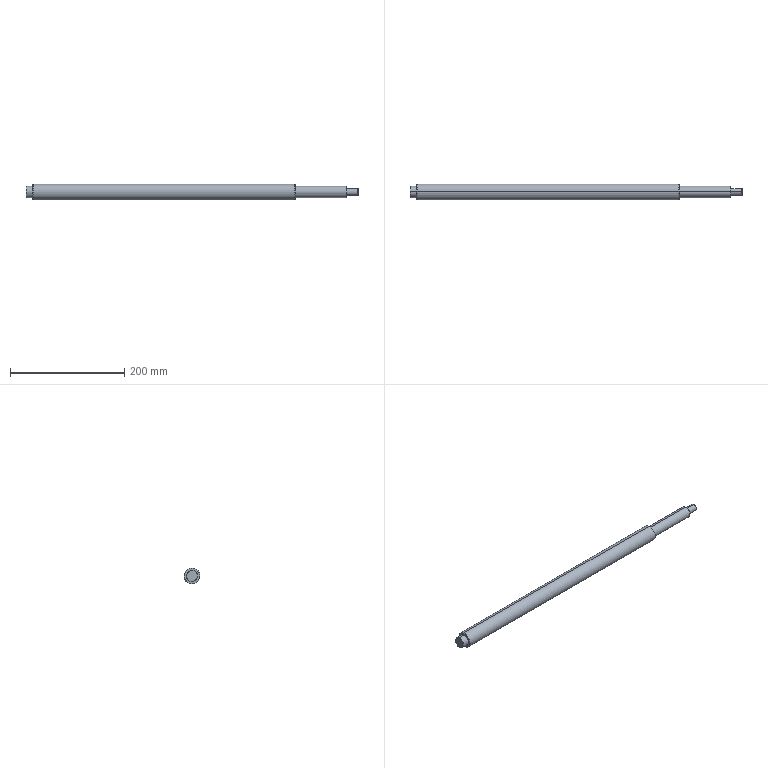Component | SolidWorks | TC020.05-03-1 | 1 solid | 34 faces | box 582 x 28 x 28 mm | volume 317223 mm3 | cone 13 | cylinder 13 | plane 8 | commonest cylinder face diameters 20 x4 12 x3 3.3 x2 28 x2 4 x2 | material 45 Steel
STEP:
#1=COLOUR_RGB('',0.7922,0.8196,0.9333);
#2=FILL_AREA_STYLE_COLOUR('',#1);
#3=FILL_AREA_STYLE('',(#2));
#4=SURFACE_STYLE_FILL_AREA(#3);
#5=SURFACE_SIDE_STYLE('',(#4));
#6=SURFACE_STYLE_USAGE(.BOTH.,#5);
#7=PRESENTATION_STYLE_ASSIGNMENT((#6));
#8=CARTESIAN_POINT('',(0.1969,1.219,0.3721));
#9=VERTEX_POINT('',#8);
#10=CARTESIAN_POINT('',(0.1969,1.143,-0.3721));
#11=VERTEX_POINT('',#10);
#12=CARTESIAN_POINT('',(0.1969,1.181,0.));
#13=DIRECTION('',(-1.,-0.,0.));
#14=DIRECTION('',(0.,0.1006,0.9949));
#15=AXIS2_PLACEMENT_3D('',#12,#13,#14);
#16=CIRCLE('',#15,0.374);
#17=EDGE_CURVE('',#9,#11,#16,.T.);
#18=ORIENTED_EDGE('',*,*,#17,.F.);
#19=CARTESIAN_POINT('',(0.2165,1.221,0.3917));
#20=VERTEX_POINT('',#19);
#21=CARTESIAN_POINT('',(0.2165,1.221,0.3917));
#22=DIRECTION('',(0.7071,0.07111,0.7035));
#23=VECTOR('',#22,39.37);
#24=LINE('',#21,#23);
#25=EDGE_CURVE('',#9,#20,#24,.T.);
#26=ORIENTED_EDGE('',*,*,#25,.T.);
#27=CARTESIAN_POINT('',(0.2165,1.142,-0.3917));
#28=VERTEX_POINT('',#27);
#29=CARTESIAN_POINT('',(0.2165,1.181,0.));
#30=DIRECTION('',(1.,0.,-0.));
#31=DIRECTION('',(0.,0.1006,0.9949));
#32=AXIS2_PLACEMENT_3D('',#29,#30,#31);
#33=CIRCLE('',#32,0.3937);
#34=EDGE_CURVE('',#28,#20,#33,.T.);
#35=ORIENTED_EDGE('',*,*,#34,.F.);
#36=CARTESIAN_POINT('',(0.2165,1.142,-0.3917));
#37=DIRECTION('',(0.7071,-0.07111,-0.7035));
#38=VECTOR('',#37,39.37);
#39=LINE('',#36,#38);
#40=EDGE_CURVE('',#11,#28,#39,.T.);
#41=ORIENTED_EDGE('',*,*,#40,.F.);
#42=EDGE_LOOP('',(#18,#26,#35,#41));
#43=FACE_OUTER_BOUND('',#42,.T.);
#44=CARTESIAN_POINT('',(0.2165,1.181,0.));
#45=DIRECTION('',(1.,0.,-0.));
#46=DIRECTION('',(-0.,-0.1006,-0.9949));
#47=AXIS2_PLACEMENT_3D('',#44,#45,#46);
#48=CONICAL_SURFACE('',#47,0.3937,0.7854);
#49=ADVANCED_FACE('',(#43),#48,.T.);
#50=CARTESIAN_POINT('',(0.6693,1.235,0.5288));
#51=VERTEX_POINT('',#50);
#52=CARTESIAN_POINT('',(0.6693,1.128,-0.5288));
#53=VERTEX_POINT('',#52);
#54=CARTESIAN_POINT('',(0.6693,1.181,0.));
#55=DIRECTION('',(-1.,-0.,0.));
#56=DIRECTION('',(0.,0.1006,0.9949));
#57=AXIS2_PLACEMENT_3D('',#54,#55,#56);
#58=CIRCLE('',#57,0.5315);
#59=EDGE_CURVE('',#51,#53,#58,.T.);
#60=ORIENTED_EDGE('',*,*,#59,.F.);
#61=CARTESIAN_POINT('',(0.689,1.237,0.5484));
#62=VERTEX_POINT('',#61);
#63=CARTESIAN_POINT('',(0.689,1.237,0.5484));
#64=DIRECTION('',(0.7071,0.07111,0.7035));
#65=VECTOR('',#64,39.37);
#66=LINE('',#63,#65);
#67=EDGE_CURVE('',#51,#62,#66,.T.);
#68=ORIENTED_EDGE('',*,*,#67,.T.);
#69=CARTESIAN_POINT('',(0.689,1.126,-0.5484));
#70=VERTEX_POINT('',#69);
#71=CARTESIAN_POINT('',(0.689,1.181,0.));
#72=DIRECTION('',(1.,0.,-0.));
#73=DIRECTION('',(0.,0.1006,0.9949));
#74=AXIS2_PLACEMENT_3D('',#71,#72,#73);
#75=CIRCLE('',#74,0.5512);
#76=EDGE_CURVE('',#70,#62,#75,.T.);
#77=ORIENTED_EDGE('',*,*,#76,.F.);
#78=CARTESIAN_POINT('',(0.689,1.126,-0.5484));
#79=DIRECTION('',(0.7071,-0.07111,-0.7035));
#80=VECTOR('',#79,39.37);
#81=LINE('',#78,#80);
#82=EDGE_CURVE('',#53,#70,#81,.T.);
#83=ORIENTED_EDGE('',*,*,#82,.F.);
#84=EDGE_LOOP('',(#60,#68,#77,#83));
#85=FACE_OUTER_BOUND('',#84,.T.);
#86=CARTESIAN_POINT('',(0.689,1.181,0.));
#87=DIRECTION('',(1.,0.,-0.));
#88=DIRECTION('',(0.,-0.1006,-0.9949));
#89=AXIS2_PLACEMENT_3D('',#86,#87,#88);
#90=CONICAL_SURFACE('',#89,0.5512,0.7854);
#91=ADVANCED_FACE('',(#85),#90,.T.);
#92=CARTESIAN_POINT('',(22.323,1.143,-0.3721));
#93=VERTEX_POINT('',#92);
#94=CARTESIAN_POINT('',(22.323,1.219,0.3721));
#95=VERTEX_POINT('',#94);
#96=CARTESIAN_POINT('',(22.323,1.181,-0.));
#97=DIRECTION('',(1.,0.,-0.));
#98=DIRECTION('',(0.,-0.1006,-0.9949));
#99=AXIS2_PLACEMENT_3D('',#96,#97,#98);
#100=CIRCLE('',#99,0.374);
#101=EDGE_CURVE('',#93,#95,#100,.T.);
#102=ORIENTED_EDGE('',*,*,#101,.F.);
#103=CARTESIAN_POINT('',(22.303,1.142,-0.3917));
#104=VERTEX_POINT('',#103);
#105=CARTESIAN_POINT('',(22.323,1.143,-0.3721));
#106=DIRECTION('',(-0.7071,-0.07111,-0.7035));
#107=VECTOR('',#106,39.37);
#108=LINE('',#105,#107);
#109=EDGE_CURVE('',#93,#104,#108,.T.);
#110=ORIENTED_EDGE('',*,*,#109,.T.);
#111=CARTESIAN_POINT('',(22.303,1.221,0.3917));
#112=VERTEX_POINT('',#111);
#113=CARTESIAN_POINT('',(22.303,1.181,-0.));
#114=DIRECTION('',(-1.,-0.,0.));
#115=DIRECTION('',(0.,-0.1006,-0.9949));
#116=AXIS2_PLACEMENT_3D('',#113,#114,#115);
#117=CIRCLE('',#116,0.3937);
#118=EDGE_CURVE('',#112,#104,#117,.T.);
#119=ORIENTED_EDGE('',*,*,#118,.F.);
#120=CARTESIAN_POINT('',(22.323,1.219,0.3721));
#121=DIRECTION('',(-0.7071,0.07111,0.7035));
#122=VECTOR('',#121,39.37);
#123=LINE('',#120,#122);
#124=EDGE_CURVE('',#95,#112,#123,.T.);
#125=ORIENTED_EDGE('',*,*,#124,.F.);
#126=EDGE_LOOP('',(#102,#110,#119,#125));
#127=FACE_OUTER_BOUND('',#126,.T.);
#128=CARTESIAN_POINT('',(22.323,1.181,-0.));
#129=DIRECTION('',(-1.,-0.,0.));
#130=DIRECTION('',(0.,0.1006,0.9949));
#131=AXIS2_PLACEMENT_3D('',#128,#129,#130);
#132=CONICAL_SURFACE('',#131,0.374,0.7854);
#133=ADVANCED_FACE('',(#127),#132,.T.);
#134=CARTESIAN_POINT('',(18.78,1.128,-0.5288));
#135=VERTEX_POINT('',#134);
#136=CARTESIAN_POINT('',(18.78,1.235,0.5288));
#137=VERTEX_POINT('',#136);
#138=CARTESIAN_POINT('',(18.78,1.181,-0.));
#139=DIRECTION('',(1.,0.,-0.));
#140=DIRECTION('',(0.,-0.1006,-0.9949));
#141=AXIS2_PLACEMENT_3D('',#138,#139,#140);
#142=CIRCLE('',#141,0.5315);
#143=EDGE_CURVE('',#135,#137,#142,.T.);
#144=ORIENTED_EDGE('',*,*,#143,.F.);
#145=CARTESIAN_POINT('',(18.76,1.126,-0.5484));
#146=VERTEX_POINT('',#145);
#147=CARTESIAN_POINT('',(18.78,1.128,-0.5288));
#148=DIRECTION('',(-0.7071,-0.07111,-0.7035));
#149=VECTOR('',#148,39.37);
#150=LINE('',#147,#149);
#151=EDGE_CURVE('',#135,#146,#150,.T.);
#152=ORIENTED_EDGE('',*,*,#151,.T.);
#153=CARTESIAN_POINT('',(18.76,1.237,0.5484));
#154=VERTEX_POINT('',#153);
#155=CARTESIAN_POINT('',(18.76,1.181,-0.));
#156=DIRECTION('',(-1.,-0.,0.));
#157=DIRECTION('',(0.,-0.1006,-0.9949));
#158=AXIS2_PLACEMENT_3D('',#155,#156,#157);
#159=CIRCLE('',#158,0.5512);
#160=EDGE_CURVE('',#154,#146,#159,.T.);
#161=ORIENTED_EDGE('',*,*,#160,.F.);
#162=CARTESIAN_POINT('',(18.78,1.235,0.5288));
#163=DIRECTION('',(-0.7071,0.07111,0.7035));
#164=VECTOR('',#163,39.37);
#165=LINE('',#162,#164);
#166=EDGE_CURVE('',#137,#154,#165,.T.);
#167=ORIENTED_EDGE('',*,*,#166,.F.);
#168=EDGE_LOOP('',(#144,#152,#161,#167));
#169=FACE_OUTER_BOUND('',#168,.T.);
#170=CARTESIAN_POINT('',(18.78,1.181,-0.));
#171=DIRECTION('',(-1.,-0.,0.));
#172=DIRECTION('',(0.,0.1006,0.9949));
#173=AXIS2_PLACEMENT_3D('',#170,#171,#172);
#174=CONICAL_SURFACE('',#173,0.5315,0.7854);
#175=ADVANCED_FACE('',(#169),#174,.T.);
#176=CARTESIAN_POINT('',(23.11,1.159,-0.2154));
#177=VERTEX_POINT('',#176);
#178=CARTESIAN_POINT('',(23.11,1.374,-0.09863));
#179=VERTEX_POINT('',#178);
#180=CARTESIAN_POINT('',(23.11,1.181,-0.));
#181=DIRECTION('',(1.,0.,-0.));
#182=DIRECTION('',(0.,-0.1006,-0.9949));
#183=AXIS2_PLACEMENT_3D('',#180,#181,#182);
#184=CIRCLE('',#183,0.2165);
#185=EDGE_CURVE('',#177,#179,#184,.T.);
#186=ORIENTED_EDGE('',*,*,#185,.F.);
#187=CARTESIAN_POINT('',(23.091,1.157,-0.235));
#188=VERTEX_POINT('',#187);
#189=CARTESIAN_POINT('',(23.11,1.159,-0.2154));
#190=DIRECTION('',(-0.7071,-0.07111,-0.7035));
#191=VECTOR('',#190,39.37);
#192=LINE('',#189,#191);
#193=EDGE_CURVE('',#177,#188,#192,.T.);
#194=ORIENTED_EDGE('',*,*,#193,.T.);
#195=CARTESIAN_POINT('',(23.091,1.395,-0.1007));
#196=VERTEX_POINT('',#195);
#197=CARTESIAN_POINT('',(23.091,1.181,-0.));
#198=DIRECTION('',(-1.,-0.,0.));
#199=DIRECTION('',(0.,-0.1006,-0.9949));
#200=AXIS2_PLACEMENT_3D('',#197,#198,#199);
#201=CIRCLE('',#200,0.2362);
#202=EDGE_CURVE('',#196,#188,#201,.T.);
#203=ORIENTED_EDGE('',*,*,#202,.F.);
#204=CARTESIAN_POINT('',(23.11,1.374,-0.09863));
#205=CARTESIAN_POINT('',(23.104,1.381,-0.09933));
#206=CARTESIAN_POINT('',(23.097,1.388,-0.1));
#207=CARTESIAN_POINT('',(23.091,1.395,-0.1007));
#208=B_SPLINE_CURVE_WITH_KNOTS('',3,(#204,#205,#206,#207),.UNSPECIFIED.,.F.,.F.,(4,4),(0.,0.0007311),.UNSPECIFIED.);
#209=EDGE_CURVE('',#179,#196,#208,.T.);
#210=ORIENTED_EDGE('',*,*,#209,.F.);
#211=EDGE_LOOP('',(#186,#194,#203,#210));
#212=FACE_OUTER_BOUND('',#211,.T.);
#213=CARTESIAN_POINT('',(23.11,1.181,-0.));
#214=DIRECTION('',(-1.,-0.,0.));
#215=DIRECTION('',(0.,0.1006,0.9949));
#216=AXIS2_PLACEMENT_3D('',#213,#214,#215);
#217=CONICAL_SURFACE('',#216,0.2165,0.7854);
#218=ADVANCED_FACE('',(#212),#217,.T.);
#219=ORIENTED_EDGE('',*,*,#193,.F.);
#220=CARTESIAN_POINT('',(23.11,1.203,0.2154));
#221=VERTEX_POINT('',#220);
#222=CARTESIAN_POINT('',(23.11,1.181,-0.));
#223=DIRECTION('',(1.,0.,-0.));
#224=DIRECTION('',(0.,-0.1006,-0.9949));
#225=AXIS2_PLACEMENT_3D('',#222,#223,#224);
#226=CIRCLE('',#225,0.2165);
#227=EDGE_CURVE('',#221,#177,#226,.T.);
#228=ORIENTED_EDGE('',*,*,#227,.F.);
#229=CARTESIAN_POINT('',(23.091,1.205,0.235));
#230=VERTEX_POINT('',#229);
#231=CARTESIAN_POINT('',(23.11,1.203,0.2154));
#232=DIRECTION('',(-0.7071,0.07111,0.7035));
#233=VECTOR('',#232,39.37);
#234=LINE('',#231,#233);
#235=EDGE_CURVE('',#221,#230,#234,.T.);
#236=ORIENTED_EDGE('',*,*,#235,.T.);
#237=CARTESIAN_POINT('',(23.091,1.181,-0.));
#238=DIRECTION('',(-1.,-0.,0.));
#239=DIRECTION('',(0.,-0.1006,-0.9949));
#240=AXIS2_PLACEMENT_3D('',#237,#238,#239);
#241=CIRCLE('',#240,0.2362);
#242=EDGE_CURVE('',#188,#230,#241,.T.);
#243=ORIENTED_EDGE('',*,*,#242,.F.);
#244=EDGE_LOOP('',(#219,#228,#236,#243));
#245=FACE_OUTER_BOUND('',#244,.T.);
#246=CARTESIAN_POINT('',(23.11,1.181,-0.));
#247=DIRECTION('',(-1.,-0.,0.));
#248=DIRECTION('',(0.,0.1006,0.9949));
#249=AXIS2_PLACEMENT_3D('',#246,#247,#248);
#250=CONICAL_SURFACE('',#249,0.2165,0.7854);
#251=ADVANCED_FACE('',(#245),#250,.T.);
#252=CARTESIAN_POINT('',(22.657,1.188,0.06463));
#253=VERTEX_POINT('',#252);
#254=CARTESIAN_POINT('',(22.657,1.175,-0.06463));
#255=VERTEX_POINT('',#254);
#256=CARTESIAN_POINT('',(22.657,1.181,-0.));
#257=DIRECTION('',(1.,0.,-0.));
#258=DIRECTION('',(0.,-0.1006,-0.9949));
#259=AXIS2_PLACEMENT_3D('',#256,#257,#258);
#260=CIRCLE('',#259,0.06496);
#261=EDGE_CURVE('',#253,#255,#260,.T.);
#262=ORIENTED_EDGE('',*,*,#261,.F.);
#263=CARTESIAN_POINT('',(23.11,1.188,0.06463));
#264=VERTEX_POINT('',#263);
#265=CARTESIAN_POINT('',(23.11,1.188,0.06463));
#266=DIRECTION('',(1.,0.,-0.));
#267=VECTOR('',#266,39.37);
#268=LINE('',#265,#267);
#269=EDGE_CURVE('',#253,#264,#268,.T.);
#270=ORIENTED_EDGE('',*,*,#269,.T.);
#271=CARTESIAN_POINT('',(23.11,1.175,-0.06463));
#272=VERTEX_POINT('',#271);
#273=CARTESIAN_POINT('',(23.11,1.181,-0.));
#274=DIRECTION('',(1.,0.,-0.));
#275=DIRECTION('',(0.,-0.1006,-0.9949));
#276=AXIS2_PLACEMENT_3D('',#273,#274,#275);
#277=CIRCLE('',#276,0.06496);
#278=EDGE_CURVE('',#264,#272,#277,.T.);
#279=ORIENTED_EDGE('',*,*,#278,.T.);
#280=CARTESIAN_POINT('',(23.11,1.175,-0.06463));
#281=DIRECTION('',(1.,0.,-0.));
#282=VECTOR('',#281,39.37);
#283=LINE('',#280,#282);
#284=EDGE_CURVE('',#255,#272,#283,.T.);
#285=ORIENTED_EDGE('',*,*,#284,.F.);
#286=EDGE_LOOP('',(#262,#270,#279,#285));
#287=FACE_OUTER_BOUND('',#286,.T.);
#288=CARTESIAN_POINT('',(23.11,1.181,-0.));
#289=DIRECTION('',(1.,0.,-0.));
#290=DIRECTION('',(0.,-0.1006,-0.9949));
#291=AXIS2_PLACEMENT_3D('',#288,#289,#290);
#292=CYLINDRICAL_SURFACE('',#291,0.06496);
#293=ADVANCED_FACE('',(#287),#292,.F.);
#294=CARTESIAN_POINT('',(22.618,1.181,-0.));
#295=VERTEX_POINT('',#294);
#296=CARTESIAN_POINT('',(22.657,1.175,-0.06463));
#297=DIRECTION('',(0.515,-0.08621,-0.8528));
#298=VECTOR('',#297,39.37);
#299=LINE('',#296,#298);
#300=EDGE_CURVE('',#295,#255,#299,.T.);
#301=ORIENTED_EDGE('',*,*,#300,.F.);
#302=CARTESIAN_POINT('',(22.657,1.188,0.06463));
#303=DIRECTION('',(0.515,0.08621,0.8528));
#304=VECTOR('',#303,39.37);
#305=LINE('',#302,#304);
#306=EDGE_CURVE('',#295,#253,#305,.T.);
#307=ORIENTED_EDGE('',*,*,#306,.T.);
#308=ORIENTED_EDGE('',*,*,#261,.T.);
#309=EDGE_LOOP('',(#301,#307,#308));
#310=FACE_OUTER_BOUND('',#309,.T.);
#311=CARTESIAN_POINT('',(22.657,1.181,-0.));
#312=DIRECTION('',(1.,0.,-0.));
#313=DIRECTION('',(0.,-0.1006,-0.9949));
#314=AXIS2_PLACEMENT_3D('',#311,#312,#313);
#315=CONICAL_SURFACE('',#314,0.06496,1.03);
#316=ADVANCED_FACE('',(#310),#315,.F.);
#317=CARTESIAN_POINT('',(22.323,1.416,-0.02376));
#318=VERTEX_POINT('',#317);
#319=CARTESIAN_POINT('',(22.323,1.205,0.235));
#320=VERTEX_POINT('',#319);
#321=CARTESIAN_POINT('',(22.323,1.181,-0.));
#322=DIRECTION('',(1.,0.,-0.));
#323=DIRECTION('',(0.,-0.1006,-0.9949));
#324=AXIS2_PLACEMENT_3D('',#321,#322,#323);
#325=CIRCLE('',#324,0.2362);
#326=EDGE_CURVE('',#318,#320,#325,.T.);
#327=ORIENTED_EDGE('',*,*,#326,.T.);
#328=CARTESIAN_POINT('',(23.11,1.205,0.235));
#329=DIRECTION('',(1.,0.,-0.));
#330=VECTOR('',#329,39.37);
#331=LINE('',#328,#330);
#332=EDGE_CURVE('',#320,#230,#331,.T.);
#333=ORIENTED_EDGE('',*,*,#332,.T.);
#334=CARTESIAN_POINT('',(23.091,1.411,0.05594));
#335=VERTEX_POINT('',#334);
#336=CARTESIAN_POINT('',(23.091,1.181,-0.));
#337=DIRECTION('',(-1.,-0.,0.));
#338=DIRECTION('',(0.,-0.1006,-0.9949));
#339=AXIS2_PLACEMENT_3D('',#336,#337,#338);
#340=CIRCLE('',#339,0.2362);
#341=EDGE_CURVE('',#230,#335,#340,.T.);
#342=ORIENTED_EDGE('',*,*,#341,.T.);
#343=CARTESIAN_POINT('',(22.402,1.411,0.05594));
#344=VERTEX_POINT('',#343);
#345=CARTESIAN_POINT('',(23.11,1.411,0.05594));
#346=DIRECTION('',(1.,0.,-0.));
#347=VECTOR('',#346,39.37);
#348=LINE('',#345,#347);
#349=EDGE_CURVE('',#344,#335,#348,.T.);
#350=ORIENTED_EDGE('',*,*,#349,.F.);
#351=CARTESIAN_POINT('',(22.402,1.411,0.05594));
#352=CARTESIAN_POINT('',(22.396,1.411,0.05594));
#353=CARTESIAN_POINT('',(22.391,1.411,0.05541));
#354=CARTESIAN_POINT('',(22.381,1.411,0.05333));
#355=CARTESIAN_POINT('',(22.376,1.412,0.05175));
#356=CARTESIAN_POINT('',(22.367,1.412,0.04768));
#357=CARTESIAN_POINT('',(22.362,1.413,0.0452));
#358=CARTESIAN_POINT('',(22.354,1.414,0.03936));
#359=CARTESIAN_POINT('',(22.35,1.415,0.036));
#360=CARTESIAN_POINT('',(22.339,1.416,0.02499));
#361=CARTESIAN_POINT('',(22.333,1.417,0.01614));
#362=CARTESIAN_POINT('',(22.327,1.417,0.001848));
#363=CARTESIAN_POINT('',(22.325,1.417,-0.003168));
#364=CARTESIAN_POINT('',(22.323,1.417,-0.01338));
#365=CARTESIAN_POINT('',(22.323,1.417,-0.01854));
#366=CARTESIAN_POINT('',(22.323,1.416,-0.02376));
#367=B_SPLINE_CURVE_WITH_KNOTS('',3,(#351,#352,#353,#354,#355,#356,#357,#358,#359,#360,#361,#362,#363,#364,#365,#366),.UNSPECIFIED.,.F.,.F.,(4,2,2,2,2,2,2,4),(0.,0.0003934,0.0007868,0.00118,0.001574,0.00236,0.002754,0.003147),.UNSPECIFIED.);
#368=EDGE_CURVE('',#344,#318,#367,.T.);
#369=ORIENTED_EDGE('',*,*,#368,.T.);
#370=EDGE_LOOP('',(#327,#333,#342,#350,#369));
#371=FACE_OUTER_BOUND('',#370,.T.);
#372=CARTESIAN_POINT('',(23.11,1.181,-0.));
#373=DIRECTION('',(1.,0.,-0.));
#374=DIRECTION('',(0.,-0.1006,-0.9949));
#375=AXIS2_PLACEMENT_3D('',#372,#373,#374);
#376=CYLINDRICAL_SURFACE('',#375,0.2362);
#377=ADVANCED_FACE('',(#371),#376,.T.);
#378=ORIENTED_EDGE('',*,*,#332,.F.);
#379=CARTESIAN_POINT('',(22.323,1.157,-0.235));
#380=VERTEX_POINT('',#379);
#381=CARTESIAN_POINT('',(22.323,1.181,-0.));
#382=DIRECTION('',(1.,0.,-0.));
#383=DIRECTION('',(0.,-0.1006,-0.9949));
#384=AXIS2_PLACEMENT_3D('',#381,#382,#383);
#385=CIRCLE('',#384,0.2362);
#386=EDGE_CURVE('',#320,#380,#385,.T.);
#387=ORIENTED_EDGE('',*,*,#386,.T.);
#388=CARTESIAN_POINT('',(23.11,1.157,-0.235));
#389=DIRECTION('',(1.,0.,-0.));
#390=VECTOR('',#389,39.37);
#391=LINE('',#388,#390);
#392=EDGE_CURVE('',#380,#188,#391,.T.);
#393=ORIENTED_EDGE('',*,*,#392,.T.);
#394=ORIENTED_EDGE('',*,*,#242,.T.);
#395=EDGE_LOOP('',(#378,#387,#393,#394));
#396=FACE_OUTER_BOUND('',#395,.T.);
#397=CARTESIAN_POINT('',(23.11,1.181,-0.));
#398=DIRECTION('',(1.,0.,-0.));
#399=DIRECTION('',(0.,-0.1006,-0.9949));
#400=AXIS2_PLACEMENT_3D('',#397,#398,#399);
#401=CYLINDRICAL_SURFACE('',#400,0.2362);
#402=ADVANCED_FACE('',(#396),#401,.T.);
#403=CARTESIAN_POINT('',(18.78,1.142,-0.3917));
#404=VERTEX_POINT('',#403);
#405=CARTESIAN_POINT('',(18.78,1.221,0.3917));
#406=VERTEX_POINT('',#405);
#407=CARTESIAN_POINT('',(18.78,1.181,-0.));
#408=DIRECTION('',(1.,0.,-0.));
#409=DIRECTION('',(0.,-0.1006,-0.9949));
#410=AXIS2_PLACEMENT_3D('',#407,#408,#409);
#411=CIRCLE('',#410,0.3937);
#412=EDGE_CURVE('',#404,#406,#411,.T.);
#413=ORIENTED_EDGE('',*,*,#412,.T.);
#414=CARTESIAN_POINT('',(23.11,1.221,0.3917));
#415=DIRECTION('',(1.,0.,-0.));
#416=VECTOR('',#415,39.37);
#417=LINE('',#414,#416);
#418=EDGE_CURVE('',#406,#112,#417,.T.);
#419=ORIENTED_EDGE('',*,*,#418,.T.);
#420=ORIENTED_EDGE('',*,*,#118,.T.);
#421=CARTESIAN_POINT('',(23.11,1.142,-0.3917));
#422=DIRECTION('',(1.,0.,-0.));
#423=VECTOR('',#422,39.37);
#424=LINE('',#421,#423);
#425=EDGE_CURVE('',#404,#104,#424,.T.);
#426=ORIENTED_EDGE('',*,*,#425,.F.);
#427=EDGE_LOOP('',(#413,#419,#420,#426));
#428=FACE_OUTER_BOUND('',#427,.T.);
#429=CARTESIAN_POINT('',(23.11,1.181,-0.));
#430=DIRECTION('',(1.,0.,-0.));
#431=DIRECTION('',(0.,-0.1006,-0.9949));
#432=AXIS2_PLACEMENT_3D('',#429,#430,#431);
#433=CYLINDRICAL_SURFACE('',#432,0.3937);
#434=ADVANCED_FACE('',(#428),#433,.T.);
#435=ORIENTED_EDGE('',*,*,#76,.T.);
#436=CARTESIAN_POINT('',(23.11,1.237,0.5484));
#437=DIRECTION('',(1.,0.,-0.));
#438=VECTOR('',#437,39.37);
#439=LINE('',#436,#438);
#440=EDGE_CURVE('',#62,#154,#439,.T.);
#441=ORIENTED_EDGE('',*,*,#440,.T.);
#442=ORIENTED_EDGE('',*,*,#160,.T.);
#443=CARTESIAN_POINT('',(23.11,1.126,-0.5484));
#444=DIRECTION('',(1.,0.,-0.));
#445=VECTOR('',#444,39.37);
#446=LINE('',#443,#445);
#447=EDGE_CURVE('',#70,#146,#446,.T.);
#448=ORIENTED_EDGE('',*,*,#447,.F.);
#449=EDGE_LOOP('',(#435,#441,#442,#448));
#450=FACE_OUTER_BOUND('',#449,.T.);
#451=CARTESIAN_POINT('',(23.11,1.181,-0.));
#452=DIRECTION('',(1.,0.,-0.));
#453=DIRECTION('',(0.,-0.1006,-0.9949));
#454=AXIS2_PLACEMENT_3D('',#451,#452,#453);
#455=CYLINDRICAL_SURFACE('',#454,0.5512);
#456=ADVANCED_FACE('',(#450),#455,.T.);
#457=ORIENTED_EDGE('',*,*,#34,.T.);
#458=CARTESIAN_POINT('',(0.6693,1.221,0.3917));
#459=VERTEX_POINT('',#458);
#460=CARTESIAN_POINT('',(23.11,1.221,0.3917));
#461=DIRECTION('',(1.,0.,-0.));
#462=VECTOR('',#461,39.37);
#463=LINE('',#460,#462);
#464=EDGE_CURVE('',#20,#459,#463,.T.);
#465=ORIENTED_EDGE('',*,*,#464,.T.);
#466=CARTESIAN_POINT('',(0.6693,1.142,-0.3917));
#467=VERTEX_POINT('',#466);
#468=CARTESIAN_POINT('',(0.6693,1.181,0.));
#469=DIRECTION('',(1.,0.,-0.));
#470=DIRECTION('',(0.,-0.1006,-0.9949));
#471=AXIS2_PLACEMENT_3D('',#468,#469,#470);
#472=CIRCLE('',#471,0.3937);
#473=EDGE_CURVE('',#467,#459,#472,.T.);
#474=ORIENTED_EDGE('',*,*,#473,.F.);
#475=CARTESIAN_POINT('',(23.11,1.142,-0.3917));
#476=DIRECTION('',(1.,0.,-0.));
#477=VECTOR('',#476,39.37);
#478=LINE('',#475,#477);
#479=EDGE_CURVE('',#28,#467,#478,.T.);
#480=ORIENTED_EDGE('',*,*,#479,.F.);
#481=EDGE_LOOP('',(#457,#465,#474,#480));
#482=FACE_OUTER_BOUND('',#481,.T.);
#483=CARTESIAN_POINT('',(23.11,1.181,-0.));
#484=DIRECTION('',(1.,0.,-0.));
#485=DIRECTION('',(0.,-0.1006,-0.9949));
#486=AXIS2_PLACEMENT_3D('',#483,#484,#485);
#487=CYLINDRICAL_SURFACE('',#486,0.3937);
#488=ADVANCED_FACE('',(#482),#487,.T.);
#489=CARTESIAN_POINT('',(0.1969,1.181,0.));
#490=DIRECTION('',(-1.,-0.,0.));
#491=DIRECTION('',(0.,0.1006,0.9949));
#492=AXIS2_PLACEMENT_3D('',#489,#490,#491);
#493=CIRCLE('',#492,0.374);
#494=EDGE_CURVE('',#11,#9,#493,.T.);
#495=ORIENTED_EDGE('',*,*,#494,.T.);
#496=ORIENTED_EDGE('',*,*,#17,.T.);
#497=EDGE_LOOP('',(#495,#496));
#498=FACE_OUTER_BOUND('',#497,.T.);
#499=CARTESIAN_POINT('',(0.1969,1.181,0.));
#500=DIRECTION('',(-1.,-0.,0.));
#501=DIRECTION('',(0.,0.1006,0.9949));
#502=AXIS2_PLACEMENT_3D('',#499,#500,#501);
#503=PLANE('',#502);
#504=ADVANCED_FACE('',(#498),#503,.T.);
#505=ORIENTED_EDGE('',*,*,#464,.F.);
#506=CARTESIAN_POINT('',(0.2165,1.181,0.));
#507=DIRECTION('',(1.,0.,-0.));
#508=DIRECTION('',(0.,0.1006,0.9949));
#509=AXIS2_PLACEMENT_3D('',#506,#507,#508);
#510=CIRCLE('',#509,0.3937);
#511=EDGE_CURVE('',#20,#28,#510,.T.);
#512=ORIENTED_EDGE('',*,*,#511,.T.);
#513=ORIENTED_EDGE('',*,*,#479,.T.);
#514=CARTESIAN_POINT('',(0.6693,1.181,0.));
#515=DIRECTION('',(1.,0.,-0.));
#516=DIRECTION('',(0.,-0.1006,-0.9949));
#517=AXIS2_PLACEMENT_3D('',#514,#515,#516);
#518=CIRCLE('',#517,0.3937);
#519=EDGE_CURVE('',#459,#467,#518,.T.);
#520=ORIENTED_EDGE('',*,*,#519,.F.);
#521=EDGE_LOOP('',(#505,#512,#513,#520));
#522=FACE_OUTER_BOUND('',#521,.T.);
#523=CARTESIAN_POINT('',(23.11,1.181,-0.));
#524=DIRECTION('',(1.,0.,-0.));
#525=DIRECTION('',(0.,-0.1006,-0.9949));
#526=AXIS2_PLACEMENT_3D('',#523,#524,#525);
#527=CYLINDRICAL_SURFACE('',#526,0.3937);
#528=ADVANCED_FACE('',(#522),#527,.T.);
#529=CARTESIAN_POINT('',(0.6693,1.181,0.));
#530=DIRECTION('',(-1.,-0.,0.));
#531=DIRECTION('',(0.,0.1006,0.9949));
#532=AXIS2_PLACEMENT_3D('',#529,#530,#531);
#533=CIRCLE('',#532,0.5315);
#534=EDGE_CURVE('',#53,#51,#533,.T.);
#535=ORIENTED_EDGE('',*,*,#534,.T.);
#536=ORIENTED_EDGE('',*,*,#59,.T.);
#537=EDGE_LOOP('',(#535,#536));
#538=FACE_OUTER_BOUND('',#537,.T.);
#539=ORIENTED_EDGE('',*,*,#473,.T.);
#540=ORIENTED_EDGE('',*,*,#519,.T.);
#541=EDGE_LOOP('',(#539,#540));
#542=FACE_BOUND('',#541,.T.);
#543=CARTESIAN_POINT('',(0.6693,1.573,-0.0396));
#544=DIRECTION('',(-1.,-0.,0.));
#545=DIRECTION('',(0.,0.1006,0.9949));
#546=AXIS2_PLACEMENT_3D('',#543,#544,#545);
#547=PLANE('',#546);
#548=ADVANCED_FACE('',(#538,#542),#547,.T.);
#549=ORIENTED_EDGE('',*,*,#440,.F.);
#550=CARTESIAN_POINT('',(0.689,1.181,0.));
#551=DIRECTION('',(1.,0.,-0.));
#552=DIRECTION('',(0.,0.1006,0.9949));
#553=AXIS2_PLACEMENT_3D('',#550,#551,#552);
#554=CIRCLE('',#553,0.5512);
#555=EDGE_CURVE('',#62,#70,#554,.T.);
#556=ORIENTED_EDGE('',*,*,#555,.T.);
#557=ORIENTED_EDGE('',*,*,#447,.T.);
#558=CARTESIAN_POINT('',(18.76,1.181,-0.));
#559=DIRECTION('',(-1.,-0.,0.));
#560=DIRECTION('',(0.,-0.1006,-0.9949));
#561=AXIS2_PLACEMENT_3D('',#558,#559,#560);
#562=CIRCLE('',#561,0.5512);
#563=EDGE_CURVE('',#146,#154,#562,.T.);
#564=ORIENTED_EDGE('',*,*,#563,.T.);
#565=EDGE_LOOP('',(#549,#556,#557,#564));
#566=FACE_OUTER_BOUND('',#565,.T.);
#567=CARTESIAN_POINT('',(23.11,1.181,-0.));
#568=DIRECTION('',(1.,0.,-0.));
#569=DIRECTION('',(0.,-0.1006,-0.9949));
#570=AXIS2_PLACEMENT_3D('',#567,#568,#569);
#571=CYLINDRICAL_SURFACE('',#570,0.5512);
#572=ADVANCED_FACE('',(#566),#571,.T.);
#573=CARTESIAN_POINT('',(18.78,1.181,-0.));
#574=DIRECTION('',(1.,0.,-0.));
#575=DIRECTION('',(0.,-0.1006,-0.9949));
#576=AXIS2_PLACEMENT_3D('',#573,#574,#575);
#577=CIRCLE('',#576,0.5315);
#578=EDGE_CURVE('',#137,#135,#577,.T.);
#579=ORIENTED_EDGE('',*,*,#578,.T.);
#580=ORIENTED_EDGE('',*,*,#143,.T.);
#581=EDGE_LOOP('',(#579,#580));
#582=FACE_OUTER_BOUND('',#581,.T.);
#583=ORIENTED_EDGE('',*,*,#412,.F.);
#584=CARTESIAN_POINT('',(18.78,1.181,-0.));
#585=DIRECTION('',(1.,0.,-0.));
#586=DIRECTION('',(0.,-0.1006,-0.9949));
#587=AXIS2_PLACEMENT_3D('',#584,#585,#586);
#588=CIRCLE('',#587,0.3937);
#589=EDGE_CURVE('',#406,#404,#588,.T.);
#590=ORIENTED_EDGE('',*,*,#589,.F.);
#591=EDGE_LOOP('',(#583,#590));
#592=FACE_BOUND('',#591,.T.);
#593=CARTESIAN_POINT('',(18.78,1.729,-0.05543));
#594=DIRECTION('',(1.,0.,-0.));
#595=DIRECTION('',(-0.,-0.1006,-0.9949));
#596=AXIS2_PLACEMENT_3D('',#593,#594,#595);
#597=PLANE('',#596);
#598=ADVANCED_FACE('',(#582,#592),#597,.T.);
#599=ORIENTED_EDGE('',*,*,#418,.F.);
#600=ORIENTED_EDGE('',*,*,#589,.T.);
#601=ORIENTED_EDGE('',*,*,#425,.T.);
#602=CARTESIAN_POINT('',(22.303,1.181,-0.));
#603=DIRECTION('',(-1.,-0.,0.));
#604=DIRECTION('',(0.,-0.1006,-0.9949));
#605=AXIS2_PLACEMENT_3D('',#602,#603,#604);
#606=CIRCLE('',#605,0.3937);
#607=EDGE_CURVE('',#104,#112,#606,.T.);
#608=ORIENTED_EDGE('',*,*,#607,.T.);
#609=EDGE_LOOP('',(#599,#600,#601,#608));
#610=FACE_OUTER_BOUND('',#609,.T.);
#611=CARTESIAN_POINT('',(23.11,1.181,-0.));
#612=DIRECTION('',(1.,0.,-0.));
#613=DIRECTION('',(0.,-0.1006,-0.9949));
#614=AXIS2_PLACEMENT_3D('',#611,#612,#613);
#615=CYLINDRICAL_SURFACE('',#614,0.3937);
#616=ADVANCED_FACE('',(#610),#615,.T.);
#617=CARTESIAN_POINT('',(22.323,1.181,-0.));
#618=DIRECTION('',(1.,0.,-0.));
#619=DIRECTION('',(0.,-0.1006,-0.9949));
#620=AXIS2_PLACEMENT_3D('',#617,#618,#619);
#621=CIRCLE('',#620,0.374);
#622=EDGE_CURVE('',#95,#93,#621,.T.);
#623=ORIENTED_EDGE('',*,*,#622,.T.);
#624=ORIENTED_EDGE('',*,*,#101,.T.);
#625=EDGE_LOOP('',(#623,#624));
#626=FACE_OUTER_BOUND('',#625,.T.);
#627=ORIENTED_EDGE('',*,*,#326,.F.);
#628=CARTESIAN_POINT('',(22.323,1.181,-0.));
#629=DIRECTION('',(1.,0.,-0.));
#630=DIRECTION('',(0.,-0.1006,-0.9949));
#631=AXIS2_PLACEMENT_3D('',#628,#629,#630);
#632=CIRCLE('',#631,0.2362);
#633=EDGE_CURVE('',#380,#318,#632,.T.);
#634=ORIENTED_EDGE('',*,*,#633,.F.);
#635=ORIENTED_EDGE('',*,*,#386,.F.);
#636=EDGE_LOOP('',(#627,#634,#635));
#637=FACE_BOUND('',#636,.T.);
#638=CARTESIAN_POINT('',(22.323,1.573,-0.0396));
#639=DIRECTION('',(1.,0.,-0.));
#640=DIRECTION('',(-0.,-0.1006,-0.9949));
#641=AXIS2_PLACEMENT_3D('',#638,#639,#640);
#642=PLANE('',#641);
#643=ADVANCED_FACE('',(#626,#637),#642,.T.);
#644=ORIENTED_EDGE('',*,*,#392,.F.);
#645=ORIENTED_EDGE('',*,*,#633,.T.);
#646=CARTESIAN_POINT('',(22.402,1.395,-0.1007));
#647=VERTEX_POINT('',#646);
#648=CARTESIAN_POINT('',(22.323,1.416,-0.02376));
#649=CARTESIAN_POINT('',(22.323,1.416,-0.02897));
#650=CARTESIAN_POINT('',(22.323,1.415,-0.03407));
#651=CARTESIAN_POINT('',(22.325,1.413,-0.04406));
#652=CARTESIAN_POINT('',(22.327,1.412,-0.04901));
#653=CARTESIAN_POINT('',(22.331,1.41,-0.05835));
#654=CARTESIAN_POINT('',(22.333,1.409,-0.06276));
#655=CARTESIAN_POINT('',(22.339,1.406,-0.07109));
#656=CARTESIAN_POINT('',(22.342,1.405,-0.07498));
#657=CARTESIAN_POINT('',(22.353,1.401,-0.08547));
#658=CARTESIAN_POINT('',(22.362,1.399,-0.09111));
#659=CARTESIAN_POINT('',(22.376,1.397,-0.0968));
#660=CARTESIAN_POINT('',(22.381,1.396,-0.09828));
#661=CARTESIAN_POINT('',(22.391,1.395,-0.1002));
#662=CARTESIAN_POINT('',(22.396,1.395,-0.1007));
#663=CARTESIAN_POINT('',(22.402,1.395,-0.1007));
#664=B_SPLINE_CURVE_WITH_KNOTS('',3,(#648,#649,#650,#651,#652,#653,#654,#655,#656,#657,#658,#659,#660,#661,#662,#663),.UNSPECIFIED.,.F.,.F.,(4,2,2,2,2,2,2,4),(0.,0.0003934,0.0007868,0.00118,0.001574,0.00236,0.002754,0.003147),.UNSPECIFIED.);
#665=EDGE_CURVE('',#318,#647,#664,.T.);
#666=ORIENTED_EDGE('',*,*,#665,.T.);
#667=CARTESIAN_POINT('',(23.11,1.395,-0.1007));
#668=DIRECTION('',(-1.,-0.,0.));
#669=VECTOR('',#668,39.37);
#670=LINE('',#667,#669);
#671=EDGE_CURVE('',#196,#647,#670,.T.);
#672=ORIENTED_EDGE('',*,*,#671,.F.);
#673=ORIENTED_EDGE('',*,*,#202,.T.);
#674=EDGE_LOOP('',(#644,#645,#666,#672,#673));
#675=FACE_OUTER_BOUND('',#674,.T.);
#676=CARTESIAN_POINT('',(23.11,1.181,-0.));
#677=DIRECTION('',(1.,0.,-0.));
#678=DIRECTION('',(0.,-0.1006,-0.9949));
#679=AXIS2_PLACEMENT_3D('',#676,#677,#678);
#680=CYLINDRICAL_SURFACE('',#679,0.2362);
#681=ADVANCED_FACE('',(#675),#680,.T.);
#682=CARTESIAN_POINT('',(23.11,1.39,0.05805));
#683=VERTEX_POINT('',#682);
#684=CARTESIAN_POINT('',(23.11,1.326,0.06448));
#685=VERTEX_POINT('',#684);
#686=CARTESIAN_POINT('',(23.11,1.424,0.05458));
#687=DIRECTION('',(0.,-0.9949,0.1006));
#688=VECTOR('',#687,39.37);
#689=LINE('',#686,#688);
#690=EDGE_CURVE('',#683,#685,#689,.T.);
#691=ORIENTED_EDGE('',*,*,#690,.F.);
#692=CARTESIAN_POINT('',(23.11,1.181,-0.));
#693=DIRECTION('',(1.,0.,-0.));
#694=DIRECTION('',(0.,-0.1006,-0.9949));
#695=AXIS2_PLACEMENT_3D('',#692,#693,#694);
#696=CIRCLE('',#695,0.2165);
#697=EDGE_CURVE('',#683,#221,#696,.T.);
#698=ORIENTED_EDGE('',*,*,#697,.T.);
#699=ORIENTED_EDGE('',*,*,#227,.T.);
#700=ORIENTED_EDGE('',*,*,#185,.T.);
#701=CARTESIAN_POINT('',(23.11,1.31,-0.0922));
#702=VERTEX_POINT('',#701);
#703=CARTESIAN_POINT('',(23.11,1.431,-0.1044));
#704=DIRECTION('',(-0.,0.9949,-0.1006));
#705=VECTOR('',#704,39.37);
#706=LINE('',#703,#705);
#707=EDGE_CURVE('',#702,#179,#706,.T.);
#708=ORIENTED_EDGE('',*,*,#707,.F.);
#709=CARTESIAN_POINT('',(23.11,1.326,0.06448));
#710=DIRECTION('',(-0.,-0.1006,-0.9949));
#711=VECTOR('',#710,39.37);
#712=LINE('',#709,#711);
#713=EDGE_CURVE('',#685,#702,#712,.T.);
#714=ORIENTED_EDGE('',*,*,#713,.F.);
#715=EDGE_LOOP('',(#691,#698,#699,#700,#708,#714));
#716=FACE_OUTER_BOUND('',#715,.T.);
#717=CARTESIAN_POINT('',(23.11,1.181,-0.));
#718=DIRECTION('',(1.,0.,-0.));
#719=DIRECTION('',(0.,-0.1006,-0.9949));
#720=AXIS2_PLACEMENT_3D('',#717,#718,#719);
#721=CIRCLE('',#720,0.06496);
#722=EDGE_CURVE('',#272,#264,#721,.T.);
#723=ORIENTED_EDGE('',*,*,#722,.F.);
#724=ORIENTED_EDGE('',*,*,#278,.F.);
#725=EDGE_LOOP('',(#723,#724));
#726=FACE_BOUND('',#725,.T.);
#727=CARTESIAN_POINT('',(23.11,1.416,-0.02376));
#728=DIRECTION('',(1.,0.,-0.));
#729=DIRECTION('',(-0.,-0.1006,-0.9949));
#730=AXIS2_PLACEMENT_3D('',#727,#728,#729);
#731=PLANE('',#730);
#732=ADVANCED_FACE('',(#716,#726),#731,.T.);
#733=ORIENTED_EDGE('',*,*,#306,.F.);
#734=ORIENTED_EDGE('',*,*,#300,.T.);
#735=CARTESIAN_POINT('',(22.657,1.181,-0.));
#736=DIRECTION('',(1.,0.,-0.));
#737=DIRECTION('',(0.,-0.1006,-0.9949));
#738=AXIS2_PLACEMENT_3D('',#735,#736,#737);
#739=CIRCLE('',#738,0.06496);
#740=EDGE_CURVE('',#255,#253,#739,.T.);
#741=ORIENTED_EDGE('',*,*,#740,.T.);
#742=EDGE_LOOP('',(#733,#734,#741));
#743=FACE_OUTER_BOUND('',#742,.T.);
#744=CARTESIAN_POINT('',(22.657,1.181,-0.));
#745=DIRECTION('',(1.,0.,-0.));
#746=DIRECTION('',(0.,-0.1006,-0.9949));
#747=AXIS2_PLACEMENT_3D('',#744,#745,#746);
#748=CONICAL_SURFACE('',#747,0.06496,1.03);
#749=ADVANCED_FACE('',(#743),#748,.F.);
#750=ORIENTED_EDGE('',*,*,#269,.F.);
#751=ORIENTED_EDGE('',*,*,#740,.F.);
#752=ORIENTED_EDGE('',*,*,#284,.T.);
#753=ORIENTED_EDGE('',*,*,#722,.T.);
#754=EDGE_LOOP('',(#750,#751,#752,#753));
#755=FACE_OUTER_BOUND('',#754,.T.);
#756=CARTESIAN_POINT('',(23.11,1.181,-0.));
#757=DIRECTION('',(1.,0.,-0.));
#758=DIRECTION('',(0.,-0.1006,-0.9949));
#759=AXIS2_PLACEMENT_3D('',#756,#757,#758);
#760=CYLINDRICAL_SURFACE('',#759,0.06496);
#761=ADVANCED_FACE('',(#755),#760,.F.);
#762=ORIENTED_EDGE('',*,*,#349,.T.);
#763=CARTESIAN_POINT('',(23.091,1.411,0.05594));
#764=CARTESIAN_POINT('',(23.097,1.404,0.05664));
#765=CARTESIAN_POINT('',(23.104,1.397,0.05735));
#766=CARTESIAN_POINT('',(23.11,1.39,0.05805));
#767=B_SPLINE_CURVE_WITH_KNOTS('',3,(#763,#764,#765,#766),.UNSPECIFIED.,.F.,.F.,(4,4),(0.,0.0007311),.UNSPECIFIED.);
#768=EDGE_CURVE('',#335,#683,#767,.T.);
#769=ORIENTED_EDGE('',*,*,#768,.T.);
#770=ORIENTED_EDGE('',*,*,#690,.T.);
#771=CARTESIAN_POINT('',(22.402,1.326,0.06448));
#772=VERTEX_POINT('',#771);
#773=CARTESIAN_POINT('',(22.124,1.326,0.06448));
#774=DIRECTION('',(1.,0.,-0.));
#775=VECTOR('',#774,39.37);
#776=LINE('',#773,#775);
#777=EDGE_CURVE('',#772,#685,#776,.T.);
#778=ORIENTED_EDGE('',*,*,#777,.F.);
#779=CARTESIAN_POINT('',(22.402,1.447,0.05227));
#780=DIRECTION('',(-0.,0.9949,-0.1006));
#781=VECTOR('',#780,39.37);
#782=LINE('',#779,#781);
#783=EDGE_CURVE('',#772,#344,#782,.T.);
#784=ORIENTED_EDGE('',*,*,#783,.T.);
#785=EDGE_LOOP('',(#762,#769,#770,#778,#784));
#786=FACE_OUTER_BOUND('',#785,.T.);
#787=CARTESIAN_POINT('',(22.124,1.447,0.05227));
#788=DIRECTION('',(0.,0.1006,0.9949));
#789=DIRECTION('',(0.,-0.9949,0.1006));
#790=AXIS2_PLACEMENT_3D('',#787,#788,#789);
#791=PLANE('',#790);
#792=ADVANCED_FACE('',(#786),#791,.F.);
#793=ORIENTED_EDGE('',*,*,#707,.T.);
#794=ORIENTED_EDGE('',*,*,#209,.T.);
#795=ORIENTED_EDGE('',*,*,#671,.T.);
#796=CARTESIAN_POINT('',(22.402,1.31,-0.0922));
#797=VERTEX_POINT('',#796);
#798=CARTESIAN_POINT('',(22.402,1.431,-0.1044));
#799=DIRECTION('',(0.,-0.9949,0.1006));
#800=VECTOR('',#799,39.37);
#801=LINE('',#798,#800);
#802=EDGE_CURVE('',#647,#797,#801,.T.);
#803=ORIENTED_EDGE('',*,*,#802,.T.);
#804=CARTESIAN_POINT('',(22.124,1.31,-0.0922));
#805=DIRECTION('',(1.,0.,-0.));
#806=VECTOR('',#805,39.37);
#807=LINE('',#804,#806);
#808=EDGE_CURVE('',#797,#702,#807,.T.);
#809=ORIENTED_EDGE('',*,*,#808,.T.);
#810=EDGE_LOOP('',(#793,#794,#795,#803,#809));
#811=FACE_OUTER_BOUND('',#810,.T.);
#812=CARTESIAN_POINT('',(22.124,1.431,-0.1044));
#813=DIRECTION('',(-0.,-0.1006,-0.9949));
#814=DIRECTION('',(-0.,0.9949,-0.1006));
#815=AXIS2_PLACEMENT_3D('',#812,#813,#814);
#816=PLANE('',#815);
#817=ADVANCED_FACE('',(#811),#816,.F.);
#818=ORIENTED_EDGE('',*,*,#808,.F.);
#819=CARTESIAN_POINT('',(22.323,1.318,-0.01386));
#820=VERTEX_POINT('',#819);
#821=CARTESIAN_POINT('',(22.402,1.318,-0.01386));
#822=DIRECTION('',(-0.,0.9949,-0.1006));
#823=DIRECTION('',(0.,-0.1006,-0.9949));
#824=AXIS2_PLACEMENT_3D('',#821,#822,#823);
#825=CIRCLE('',#824,0.07874);
#826=EDGE_CURVE('',#797,#820,#825,.T.);
#827=ORIENTED_EDGE('',*,*,#826,.T.);
#828=CARTESIAN_POINT('',(22.402,1.318,-0.01386));
#829=DIRECTION('',(-0.,0.9949,-0.1006));
#830=DIRECTION('',(0.,-0.1006,-0.9949));
#831=AXIS2_PLACEMENT_3D('',#828,#829,#830);
#832=CIRCLE('',#831,0.07874);
#833=EDGE_CURVE('',#820,#772,#832,.T.);
#834=ORIENTED_EDGE('',*,*,#833,.T.);
#835=ORIENTED_EDGE('',*,*,#777,.T.);
#836=ORIENTED_EDGE('',*,*,#713,.T.);
#837=EDGE_LOOP('',(#818,#827,#834,#835,#836));
#838=FACE_OUTER_BOUND('',#837,.T.);
#839=CARTESIAN_POINT('',(22.124,1.326,0.06448));
#840=DIRECTION('',(0.,-0.9949,0.1006));
#841=DIRECTION('',(-0.,-0.1006,-0.9949));
#842=AXIS2_PLACEMENT_3D('',#839,#840,#841);
#843=PLANE('',#842);
#844=ADVANCED_FACE('',(#838),#843,.F.);
#845=CARTESIAN_POINT('',(22.323,1.573,-0.0396));
#846=DIRECTION('',(0.,-0.9949,0.1006));
#847=VECTOR('',#846,39.37);
#848=LINE('',#845,#847);
#849=EDGE_CURVE('',#318,#820,#848,.T.);
#850=ORIENTED_EDGE('',*,*,#849,.F.);
#851=ORIENTED_EDGE('',*,*,#368,.F.);
#852=ORIENTED_EDGE('',*,*,#783,.F.);
#853=ORIENTED_EDGE('',*,*,#833,.F.);
#854=EDGE_LOOP('',(#850,#851,#852,#853));
#855=FACE_OUTER_BOUND('',#854,.T.);
#856=CARTESIAN_POINT('',(22.402,1.439,-0.02607));
#857=DIRECTION('',(-0.,0.9949,-0.1006));
#858=DIRECTION('',(0.,0.1006,0.9949));
#859=AXIS2_PLACEMENT_3D('',#856,#857,#858);
#860=CYLINDRICAL_SURFACE('',#859,0.07874);
#861=ADVANCED_FACE('',(#855),#860,.F.);
#862=ORIENTED_EDGE('',*,*,#665,.F.);
#863=ORIENTED_EDGE('',*,*,#849,.T.);
#864=ORIENTED_EDGE('',*,*,#826,.F.);
#865=ORIENTED_EDGE('',*,*,#802,.F.);
#866=EDGE_LOOP('',(#862,#863,#864,#865));
#867=FACE_OUTER_BOUND('',#866,.T.);
#868=CARTESIAN_POINT('',(22.402,1.439,-0.02607));
#869=DIRECTION('',(0.,-0.9949,0.1006));
#870=DIRECTION('',(0.,-0.1006,-0.9949));
#871=AXIS2_PLACEMENT_3D('',#868,#869,#870);
#872=CYLINDRICAL_SURFACE('',#871,0.07874);
#873=ADVANCED_FACE('',(#867),#872,.F.);
#874=ORIENTED_EDGE('',*,*,#235,.F.);
#875=ORIENTED_EDGE('',*,*,#697,.F.);
#876=ORIENTED_EDGE('',*,*,#768,.F.);
#877=ORIENTED_EDGE('',*,*,#341,.F.);
#878=EDGE_LOOP('',(#874,#875,#876,#877));
#879=FACE_OUTER_BOUND('',#878,.T.);
#880=CARTESIAN_POINT('',(23.11,1.181,-0.));
#881=DIRECTION('',(-1.,-0.,0.));
#882=DIRECTION('',(0.,0.1006,0.9949));
#883=AXIS2_PLACEMENT_3D('',#880,#881,#882);
#884=CONICAL_SURFACE('',#883,0.2165,0.7854);
#885=ADVANCED_FACE('',(#879),#884,.T.);
#886=ORIENTED_EDGE('',*,*,#151,.F.);
#887=ORIENTED_EDGE('',*,*,#578,.F.);
#888=ORIENTED_EDGE('',*,*,#166,.T.);
#889=ORIENTED_EDGE('',*,*,#563,.F.);
#890=EDGE_LOOP('',(#886,#887,#888,#889));
#891=FACE_OUTER_BOUND('',#890,.T.);
#892=CARTESIAN_POINT('',(18.78,1.181,-0.));
#893=DIRECTION('',(-1.,-0.,0.));
#894=DIRECTION('',(0.,0.1006,0.9949));
#895=AXIS2_PLACEMENT_3D('',#892,#893,#894);
#896=CONICAL_SURFACE('',#895,0.5315,0.7854);
#897=ADVANCED_FACE('',(#891),#896,.T.);
#898=ORIENTED_EDGE('',*,*,#109,.F.);
#899=ORIENTED_EDGE('',*,*,#622,.F.);
#900=ORIENTED_EDGE('',*,*,#124,.T.);
#901=ORIENTED_EDGE('',*,*,#607,.F.);
#902=EDGE_LOOP('',(#898,#899,#900,#901));
#903=FACE_OUTER_BOUND('',#902,.T.);
#904=CARTESIAN_POINT('',(22.323,1.181,-0.));
#905=DIRECTION('',(-1.,-0.,0.));
#906=DIRECTION('',(0.,0.1006,0.9949));
#907=AXIS2_PLACEMENT_3D('',#904,#905,#906);
#908=CONICAL_SURFACE('',#907,0.374,0.7854);
#909=ADVANCED_FACE('',(#903),#908,.T.);
#910=ORIENTED_EDGE('',*,*,#67,.F.);
#911=ORIENTED_EDGE('',*,*,#534,.F.);
#912=ORIENTED_EDGE('',*,*,#82,.T.);
#913=ORIENTED_EDGE('',*,*,#555,.F.);
#914=EDGE_LOOP('',(#910,#911,#912,#913));
#915=FACE_OUTER_BOUND('',#914,.T.);
#916=CARTESIAN_POINT('',(0.689,1.181,0.));
#917=DIRECTION('',(1.,0.,-0.));
#918=DIRECTION('',(0.,-0.1006,-0.9949));
#919=AXIS2_PLACEMENT_3D('',#916,#917,#918);
#920=CONICAL_SURFACE('',#919,0.5512,0.7854);
#921=ADVANCED_FACE('',(#915),#920,.T.);
#922=ORIENTED_EDGE('',*,*,#25,.F.);
#923=ORIENTED_EDGE('',*,*,#494,.F.);
#924=ORIENTED_EDGE('',*,*,#40,.T.);
#925=ORIENTED_EDGE('',*,*,#511,.F.);
#926=EDGE_LOOP('',(#922,#923,#924,#925));
#927=FACE_OUTER_BOUND('',#926,.T.);
#928=CARTESIAN_POINT('',(0.2165,1.181,0.));
#929=DIRECTION('',(1.,0.,-0.));
#930=DIRECTION('',(-0.,-0.1006,-0.9949));
#931=AXIS2_PLACEMENT_3D('',#928,#929,#930);
#932=CONICAL_SURFACE('',#931,0.3937,0.7854);
#933=ADVANCED_FACE('',(#927),#932,.T.);
#934=CLOSED_SHELL('',(#49,#91,#133,#175,#218,#251,#293,#316,#377,#402,#434,#456,#488,#504,#528,#548,#572,#598,#616,#643,#681,#732,#749,#761,#792,#817,#844,#861,#873,#885,#897,#909,#921,#933));
#935=MANIFOLD_SOLID_BREP('',#934);
#936=STYLED_ITEM('',(#7),#935);
#937=PRESENTATION_LAYER_ASSIGNMENT('','',(#936));
#938=(LENGTH_UNIT()NAMED_UNIT(*)SI_UNIT($,.METRE.));
#939=LENGTH_MEASURE_WITH_UNIT(LENGTH_MEASURE(0.0254),#938);
#940=DIMENSIONAL_EXPONENTS(1.,0.,0.,0.,0.,0.,0.);
#941=(CONVERSION_BASED_UNIT('',#939)LENGTH_UNIT()NAMED_UNIT(#940));
#942=UNCERTAINTY_MEASURE_WITH_UNIT(LENGTH_MEASURE(0.00001),#941,'','');
#943=(NAMED_UNIT(*)PLANE_ANGLE_UNIT()SI_UNIT($,.RADIAN.));
#944=(NAMED_UNIT(*)SI_UNIT($,.STERADIAN.)SOLID_ANGLE_UNIT());
#945=(GEOMETRIC_REPRESENTATION_CONTEXT(3)GLOBAL_UNCERTAINTY_ASSIGNED_CONTEXT((#942))GLOBAL_UNIT_ASSIGNED_CONTEXT((#941,#943,#944))REPRESENTATION_CONTEXT('',''));
#946=MECHANICAL_DESIGN_GEOMETRIC_PRESENTATION_REPRESENTATION('',(#936),#945);
#947=CARTESIAN_POINT('',(0.,0.,0.));
#948=DIRECTION('',(0.,0.,1.));
#949=DIRECTION('',(1.,0.,0.));
#950=AXIS2_PLACEMENT_3D('',#947,#948,#949);
#951=(LENGTH_UNIT()NAMED_UNIT(*)SI_UNIT($,.METRE.));
#952=LENGTH_MEASURE_WITH_UNIT(LENGTH_MEASURE(0.0254),#951);
#953=DIMENSIONAL_EXPONENTS(1.,0.,0.,0.,0.,0.,0.);
#954=(CONVERSION_BASED_UNIT('',#952)LENGTH_UNIT()NAMED_UNIT(#953));
#955=UNCERTAINTY_MEASURE_WITH_UNIT(LENGTH_MEASURE(0.00001),#954,'','');
#956=(NAMED_UNIT(*)PLANE_ANGLE_UNIT()SI_UNIT($,.RADIAN.));
#957=(NAMED_UNIT(*)SI_UNIT($,.STERADIAN.)SOLID_ANGLE_UNIT());
#958=(GEOMETRIC_REPRESENTATION_CONTEXT(3)GLOBAL_UNCERTAINTY_ASSIGNED_CONTEXT((#955))GLOBAL_UNIT_ASSIGNED_CONTEXT((#954,#956,#957))REPRESENTATION_CONTEXT('',''));
#959=ADVANCED_BREP_SHAPE_REPRESENTATION('',(#935,#950),#958);